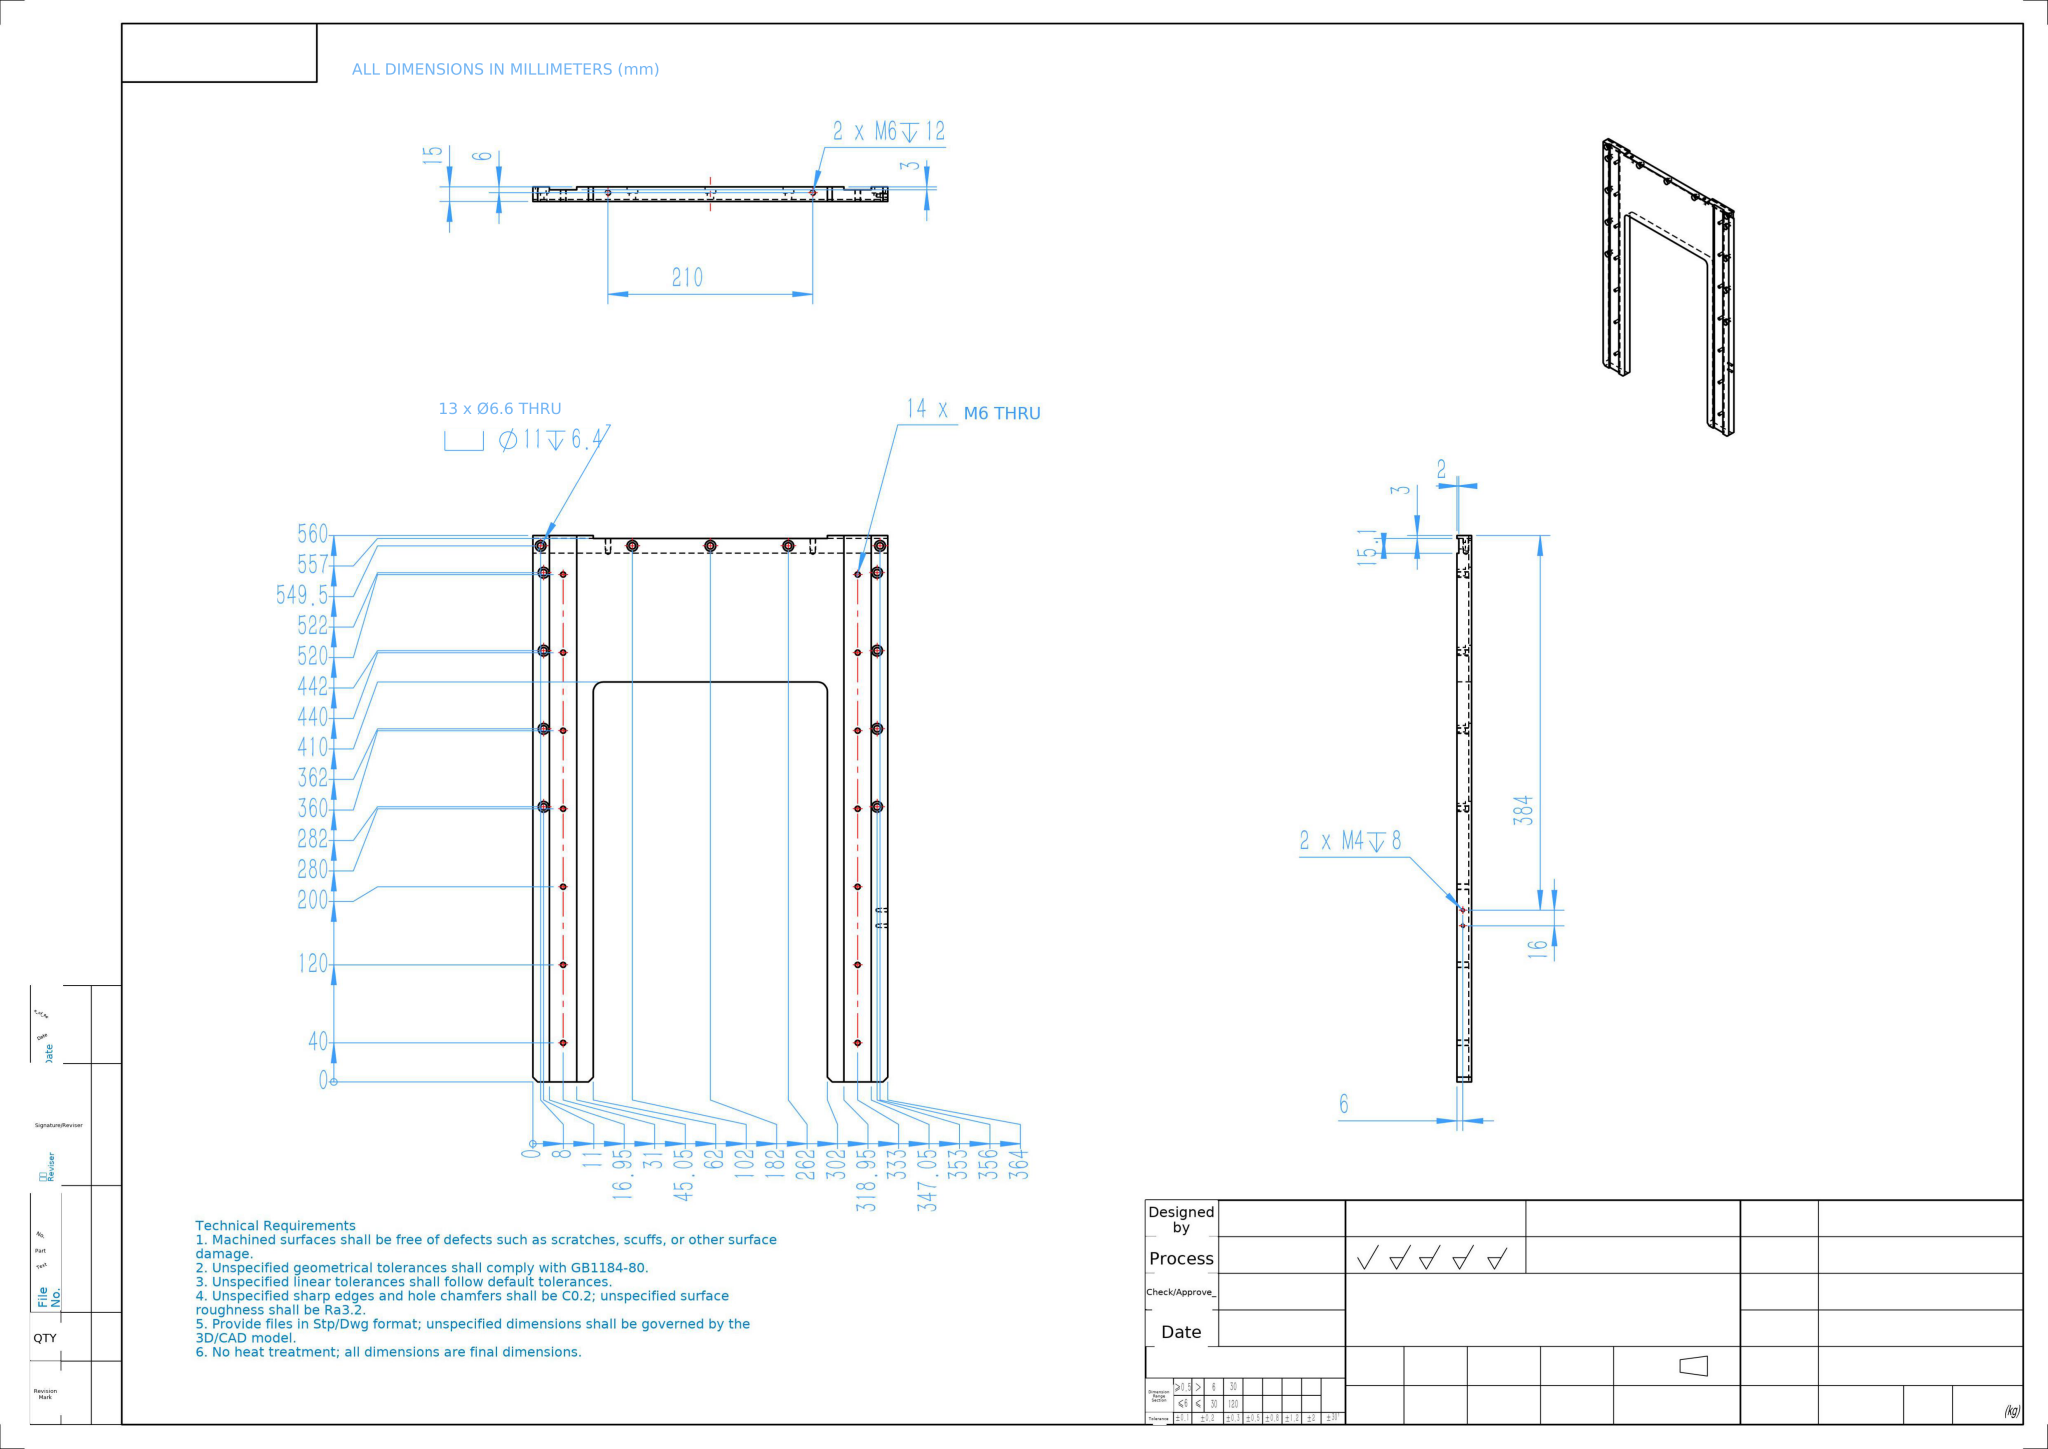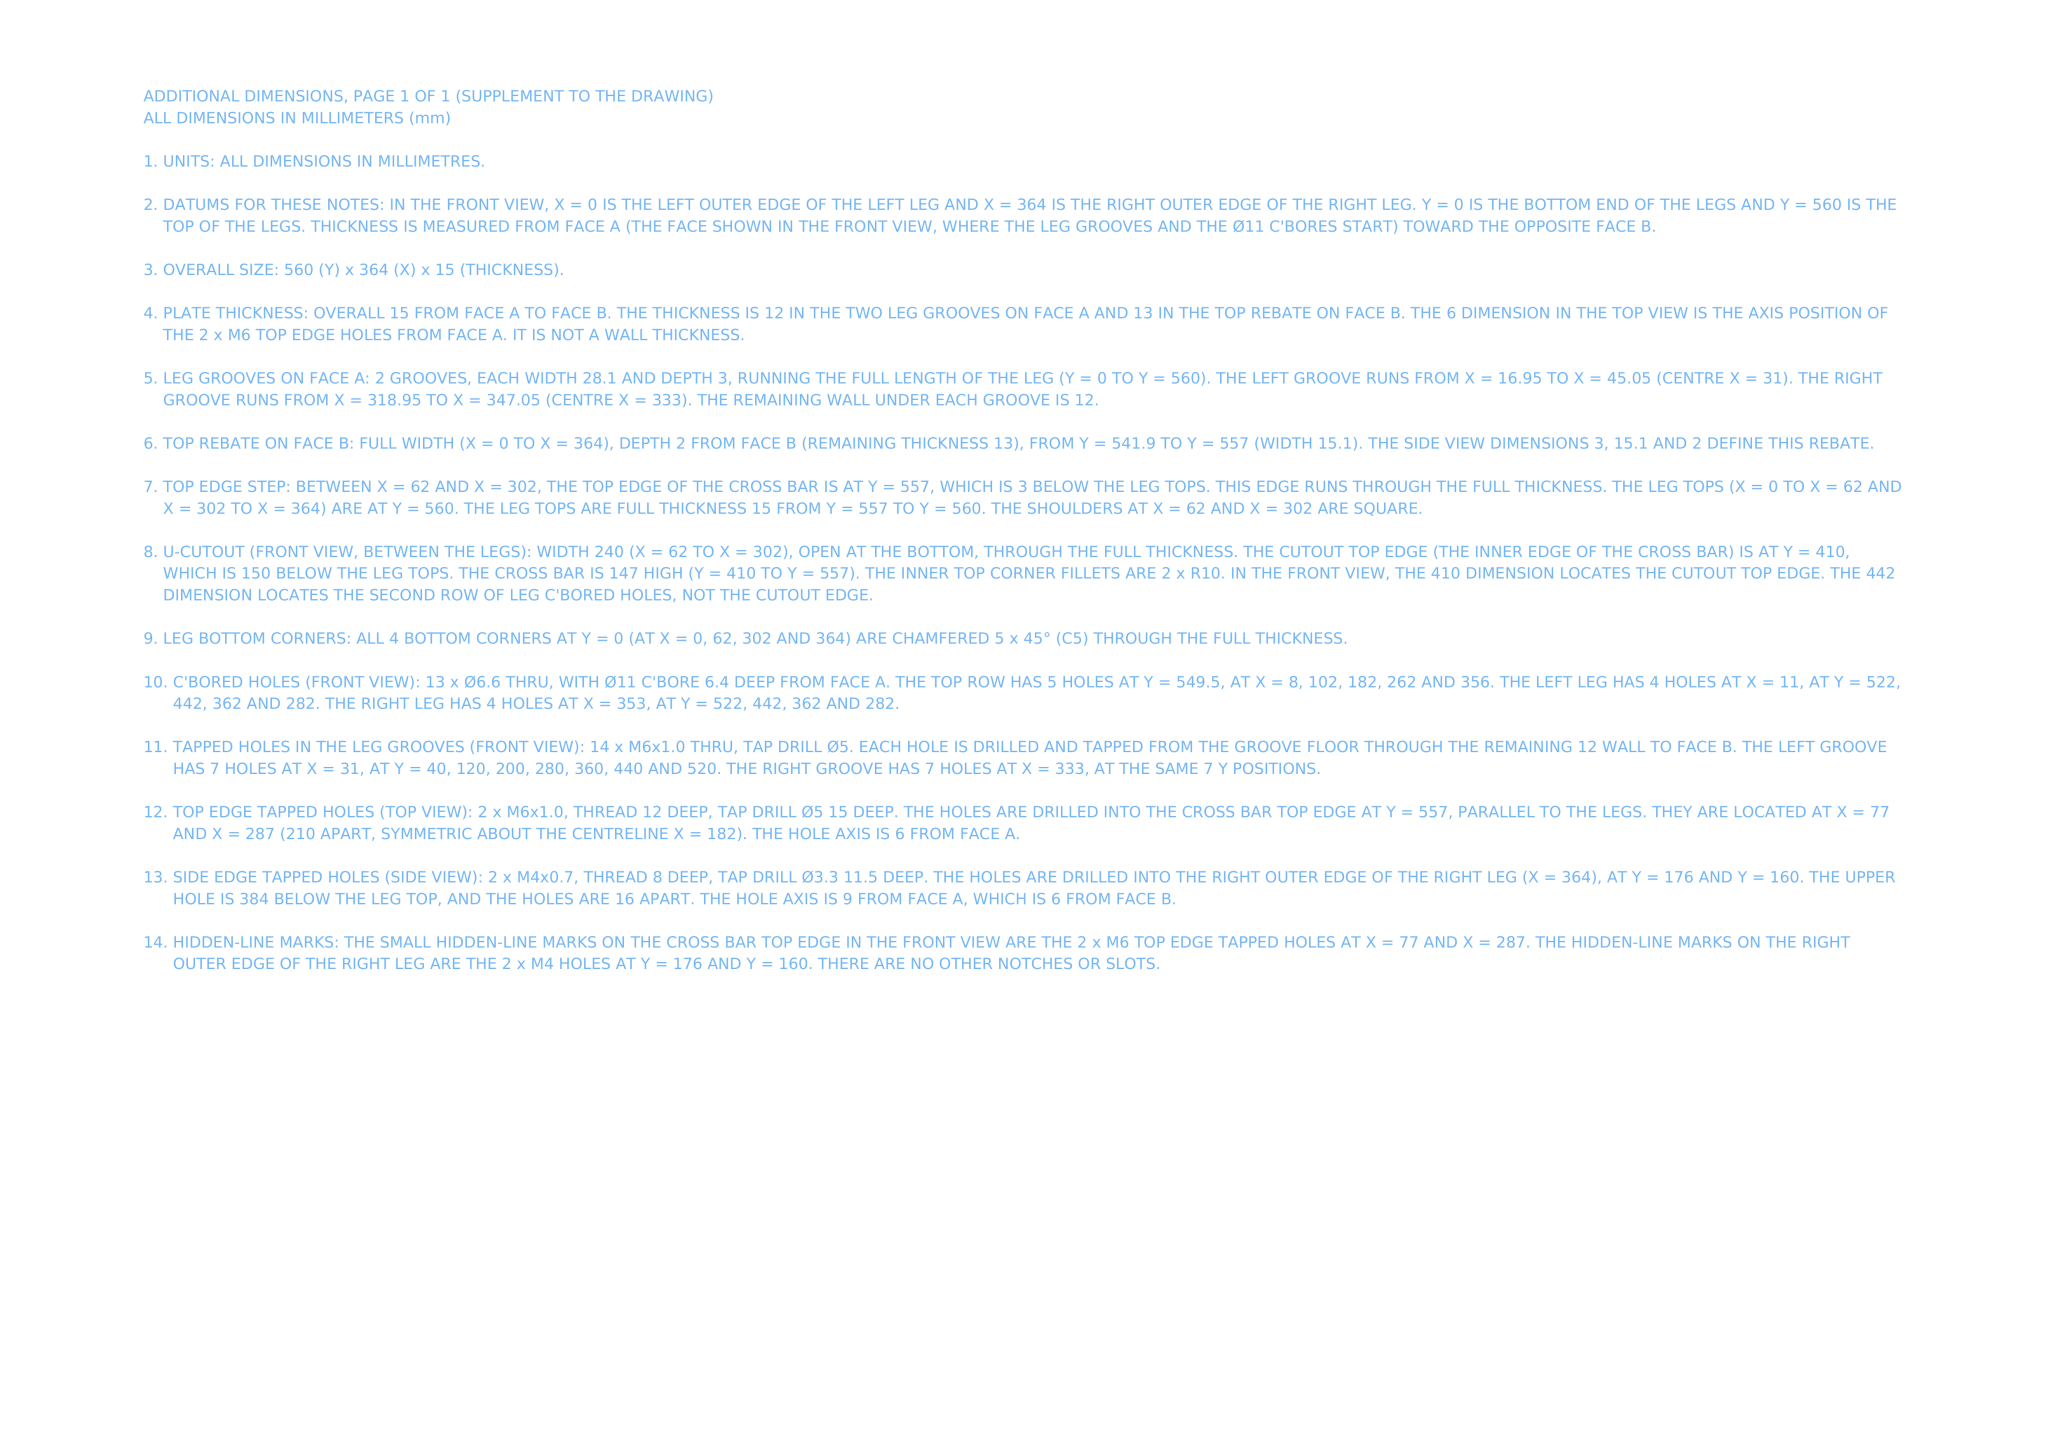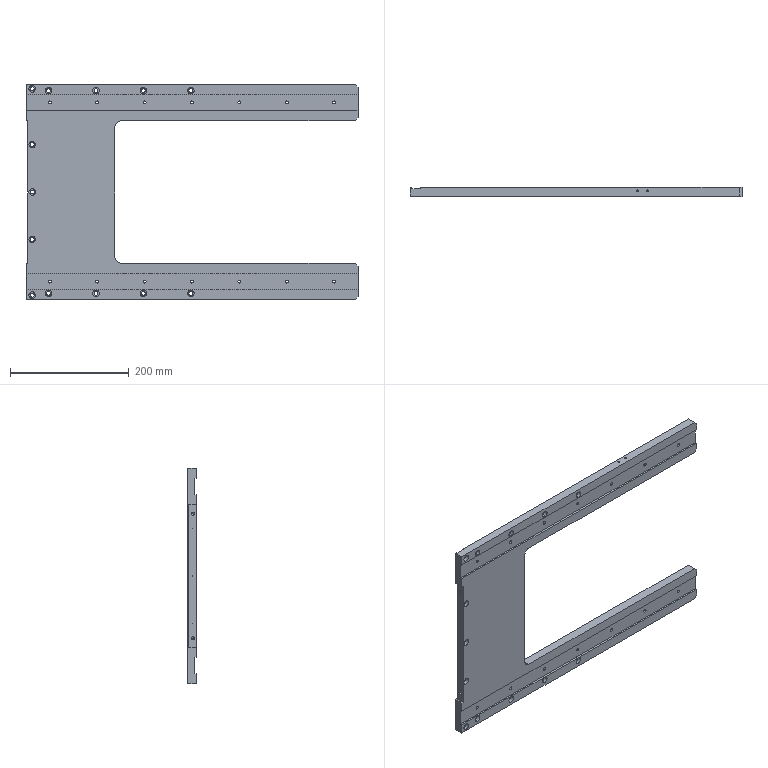Part | NX | mm | 1 solid | 143 faces | box 560 x 15 x 364 mm | volume 1449786 mm3 | cylinder 90 | plane 45 | cone 8 | commonest cylinder face diameters 5 x32 11 x26 6.6 x26 3.3 x4 20 x2